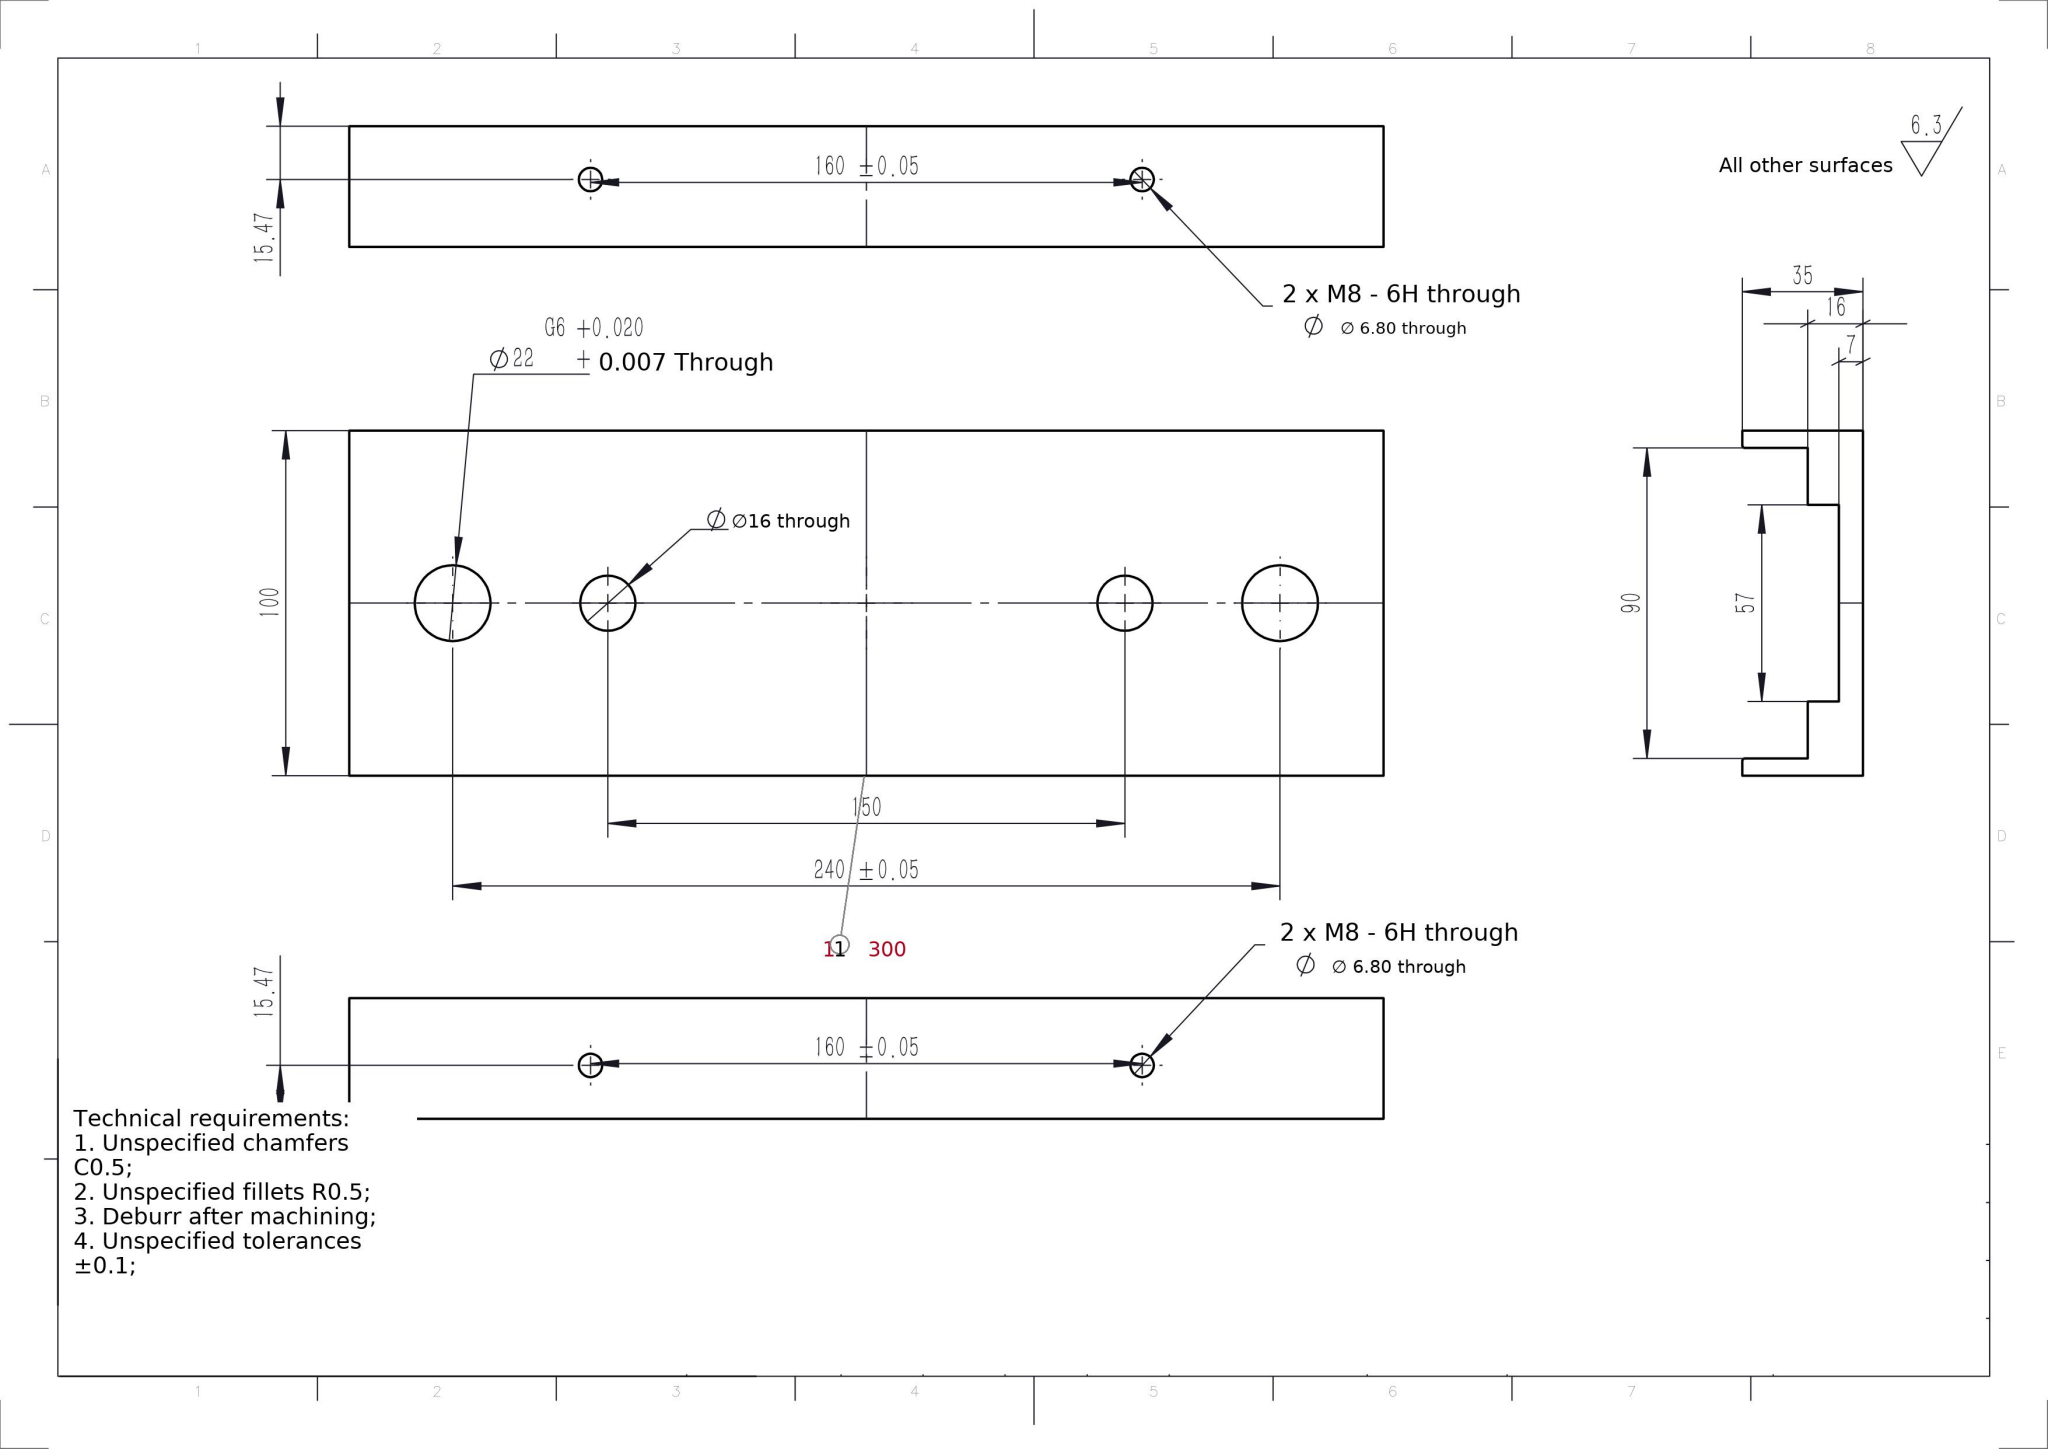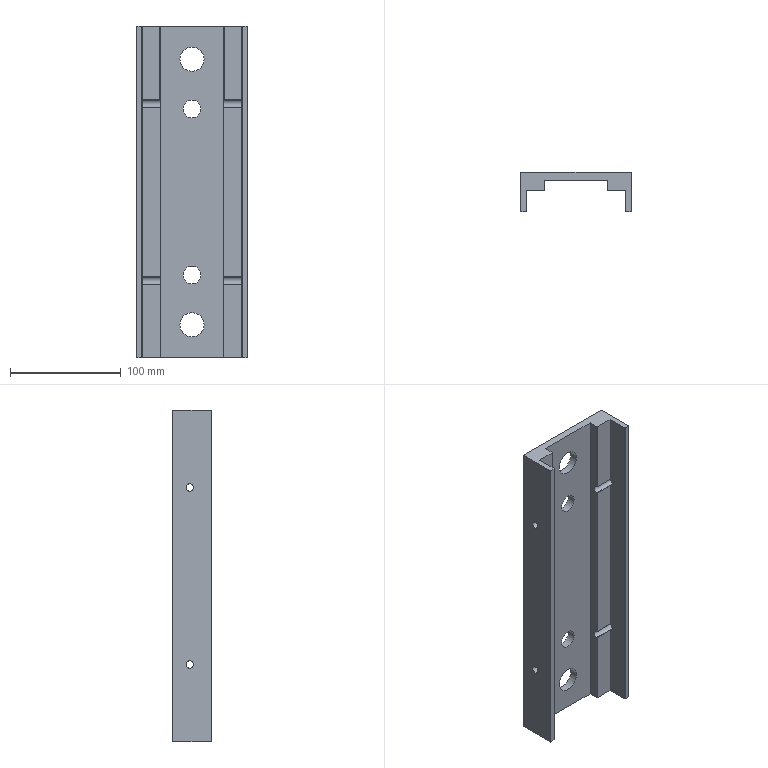Part | SolidWorks | mm | 1 solid | 38 faces | box 100 x 35 x 300 mm | volume 372711 mm3 | plane 22 | cylinder 16 | commonest cylinder face diameters 6.8 x8 22 x4 16 x4
build123d program:
from build123d import *

# Parameters (mm, degrees)
BOSS_EXTRUDE2_DEPTH = 300
SKETCH2_R           = 11
SKETCH2_R_2         = 8
CUT_EXTRUDE1_DEPTH  = 10
M8_TAPPED_HOLE1_D   = 6.8
CHAMFER1_SIZE       = 0.5


with BuildPart() as part:
    # Sketch1 → Boss-Extrude2 (new body)
    with BuildSketch(Plane.XY):
        Polygon((0, 0), (0, 35), (100, 35), (100, 0), (95, 0), (95, 19), (78.5, 19), (78.5, 28), (21.5, 28), (21.5, 19), (5, 19), (5, 0), align=None)
    extrude(amount=BOSS_EXTRUDE2_DEPTH)

    # Sketch2 → Cut-Extrude1 (cut)
    with BuildSketch(Plane(origin=(0, 35, 0), x_dir=(1, 0, 0), z_dir=(0, 1, 0))):
        with Locations(Location((50, -30, 0), (0, 0, 180))):
            Circle(SKETCH2_R)
        with Locations(Location((50, -270, 0), (0, 0, 270))):
            Circle(SKETCH2_R)
        with Locations(Location((50, -75, 0), (0, 0, 180))):
            Circle(SKETCH2_R_2)
        with Locations(Location((50, -225, 0), (0, 0, 270))):
            Circle(SKETCH2_R_2)
    extrude(amount=-CUT_EXTRUDE1_DEPTH, mode=Mode.SUBTRACT)

    # M8 Tapped Hole1 (through all)
    with Locations(Plane(origin=(100, 0, 0), x_dir=(0, 0, -1), z_dir=(1, 0, 0))):
        with Locations((-230, 19.528), (-70, 19.528)):
            Hole(M8_TAPPED_HOLE1_D / 2)

    # Chamfer1
    chamfer1_edges = [part.edges().sort_by_distance(p)[0] for p in [
        (95, 0, 150),
        (78.5, 19, 266.679),
        (21.5, 19, 266.679),
        (5, 0, 150),
    ]]
    chamfer(chamfer1_edges, length=CHAMFER1_SIZE)


solid = part.part